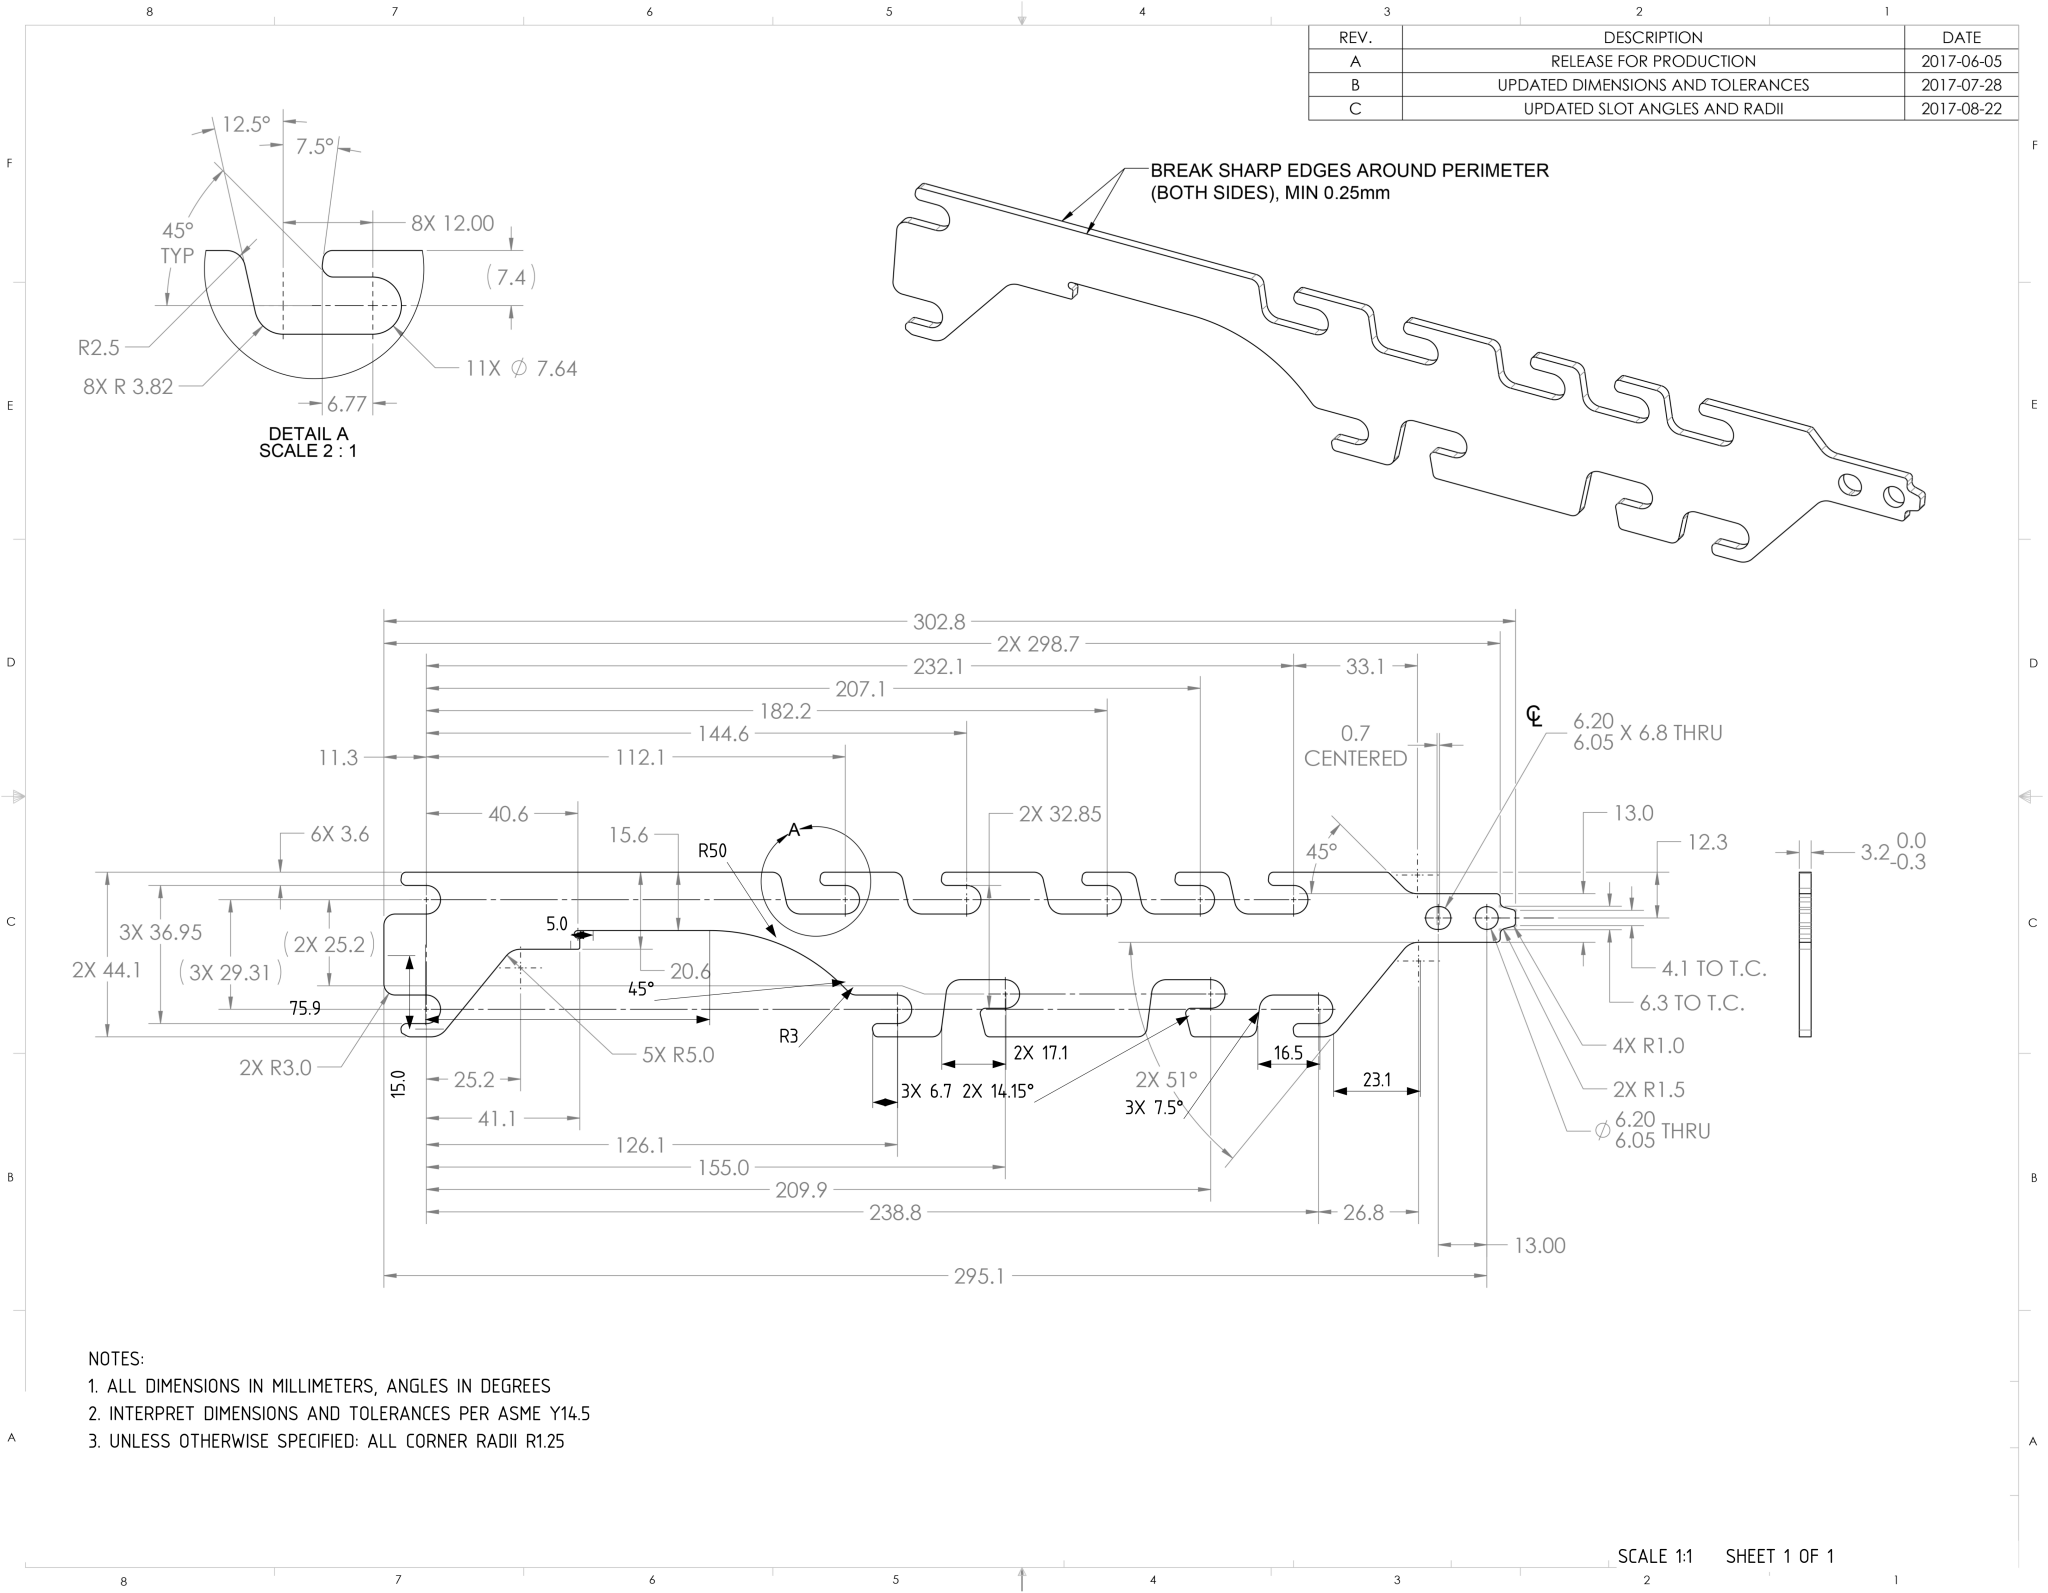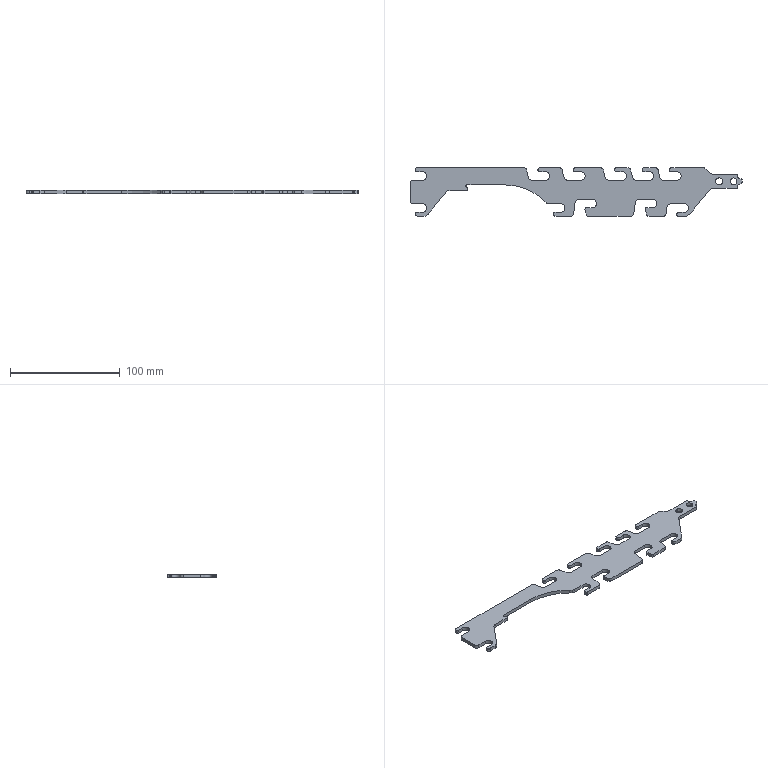Part | NX | mm | 1 solid | 180 faces | box 302.84 x 44.05 x 3.17 mm | volume 24231 mm3 | cylinder 97 | plane 83 | commonest cylinder face diameters 2.5 x43 7.644 x19 5 x8 2 x7 6.1 x5 10 x5 6 x3 3 x2